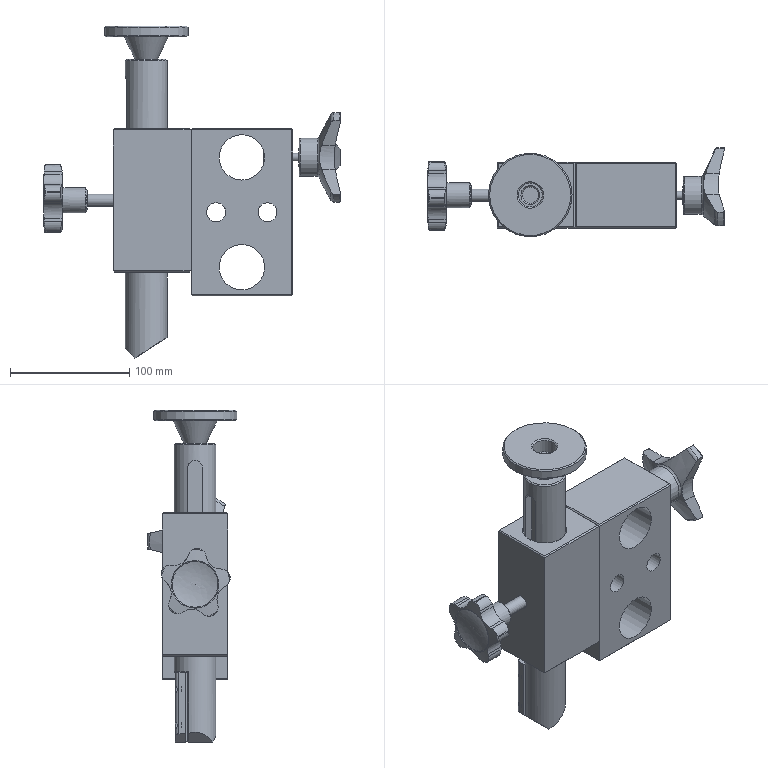Assembly | NX | mm | 6 component files | 9 solids | 243 faces | box 248.42 x 75 x 278 mm | volume 1126882 mm3 | plane 92 | cylinder 75 | cone 54 | torus 19 | spline 3 | commonest cylinder face diameters 15 x15 6.8 x6 60 x5 24.333 x5 4.5 x4 70 x4 9 x4 5 x4
Bill of materials:
unnamed part 1 | 1 |  | Three-lobed knob with a cylindrical hub, a raised circular boss on the front face, and a plain cylindrical rod sticking out of the back of the hub along its axis.
unnamed part 2 | 1 |  | Five-lobed star-shaped knob with a cylindrical hub on one side and a long, thinner cylindrical rod coming out of the hub on the same axis.
unnamed part 3 | 1 |  | Thick flat plate with a five-sided outline: three square sides and an angled, pointed end. It has four round through holes and a stepped (rabbeted) edge profile.
unnamed part 4 | 1 |  | Pin with a thin flat disc-shaped head, a conical neck under the head, and a long cylindrical shank. There is a small central hole in the head, a flat or notch near the shank tip, and an angled tip.
unnamed part 5 | 1 |  | Rectangular block with several holes: two large and two medium through holes between one pair of faces, and four counterbored holes plus one small hole on a side face.
unnamed part 6 | 1 |  | Rectangular block with one large round bore along its long axis and four small blind holes in a 2x2 pattern on one side face.
Mates:
1. center | YMSR_PET_P02 1 face | YMSR_PET_P02 1 face | YMSR_PET_P01 1 face
2. touch align | YMSR_PET_P01 1 face | YMSR_PET_P03 1 face
3. distance | YMSR_PET_P02 1 face | YMSR_PET_P01 1 face
4. parallel | YMSR_PET_P02 1 face | YMSR_PET_P01 1 edge
5. fix | YMSR_PET_P04 1 component
6. touch align | YMSR_PET_P03 1 face | YMSR_PET_P04 1 face
7. center | YMSR_PET_P03 1 face | YMSR_PET_P03 1 face | YMSR_PET_P04 1 face | YMSR_PET_P04 1 face
8. touch align | YMSR_PET_P03 1 face | YMSR_PET_P04 1 face
9. touch align | 65672_x_t 1 face | YMSR_PET_P04 1 face